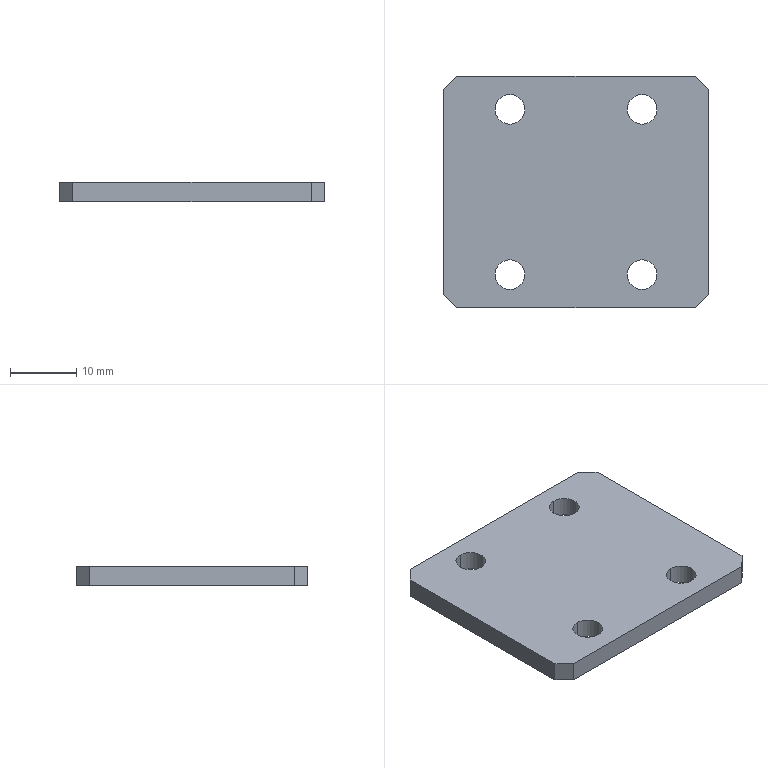Component | SolidWorks | 170423A4-RetainingPlate1-1 | 1 solid | 18 faces | box 40 x 35 x 3 mm | volume 3985 mm3 | plane 10 | cylinder 8 | commonest cylinder face diameters 4.5 x8
build123d program:
from build123d import *

# Parameters (mm, degrees)
SKETCH1_W                  = 35
SKETCH1_H                  = 40
BOSS_EXTRUDE1_DEPTH        = 3
F_4_5_4_5_DIAMETER_HOLE1_D = 4.5
CHAMFER1_SIZE              = 2


with BuildPart() as part:
    # Sketch1 → Boss-Extrude1 (new body)
    with BuildSketch(Plane.XY):
        Rectangle(SKETCH1_W, SKETCH1_H)
    extrude(amount=BOSS_EXTRUDE1_DEPTH)

    # 4.5 _4.5_ Diameter Hole1 (through all)
    with Locations(Plane.XY.offset(3)):
        with Locations((12.5, -10), (-12.5, 10), (-12.5, -10), (12.5, 10)):
            Hole(F_4_5_4_5_DIAMETER_HOLE1_D / 2)

    # Chamfer1
    chamfer1_edges = [part.edges().sort_by_distance(p)[0] for p in [
        (17.5, -20, 1.5),
        (-17.5, -20, 1.5),
        (-17.5, 20, 1.5),
        (17.5, 20, 1.5),
    ]]
    chamfer(chamfer1_edges, length=CHAMFER1_SIZE)


solid = part.part

# Placed as in the assembly
solid = solid.moved(Location((-1.246, -95.788, 406), (0, 0, 90)))
STEP:
#1=CARTESIAN_POINT('',(0.3446,-3.19,15.984));
#2=VERTEX_POINT('',#1);
#3=CARTESIAN_POINT('',(0.3446,-3.368,15.984));
#4=VERTEX_POINT('',#3);
#5=CARTESIAN_POINT('',(0.3446,-3.279,15.984));
#6=DIRECTION('',(0.,0.,1.));
#7=DIRECTION('',(0.,-1.,0.));
#8=AXIS2_PLACEMENT_3D('',#5,#6,#7);
#9=CIRCLE('',#8,0.08858);
#10=EDGE_CURVE('',#2,#4,#9,.T.);
#11=ORIENTED_EDGE('',*,*,#10,.F.);
#12=CARTESIAN_POINT('',(0.3446,-3.19,16.102));
#13=VERTEX_POINT('',#12);
#14=CARTESIAN_POINT('',(0.3446,-3.19,16.102));
#15=DIRECTION('',(0.,0.,1.));
#16=VECTOR('',#15,39.37);
#17=LINE('',#14,#16);
#18=EDGE_CURVE('',#2,#13,#17,.T.);
#19=ORIENTED_EDGE('',*,*,#18,.T.);
#20=CARTESIAN_POINT('',(0.3446,-3.368,16.102));
#21=VERTEX_POINT('',#20);
#22=CARTESIAN_POINT('',(0.3446,-3.279,16.102));
#23=DIRECTION('',(0.,0.,1.));
#24=DIRECTION('',(0.,-1.,0.));
#25=AXIS2_PLACEMENT_3D('',#22,#23,#24);
#26=CIRCLE('',#25,0.08858);
#27=EDGE_CURVE('',#13,#21,#26,.T.);
#28=ORIENTED_EDGE('',*,*,#27,.T.);
#29=CARTESIAN_POINT('',(0.3446,-3.368,16.102));
#30=DIRECTION('',(0.,0.,1.));
#31=VECTOR('',#30,39.37);
#32=LINE('',#29,#31);
#33=EDGE_CURVE('',#4,#21,#32,.T.);
#34=ORIENTED_EDGE('',*,*,#33,.F.);
#35=EDGE_LOOP('',(#11,#19,#28,#34));
#36=FACE_OUTER_BOUND('',#35,.T.);
#37=CARTESIAN_POINT('',(0.3446,-3.279,16.102));
#38=DIRECTION('',(0.,0.,1.));
#39=DIRECTION('',(0.,-1.,0.));
#40=AXIS2_PLACEMENT_3D('',#37,#38,#39);
#41=CYLINDRICAL_SURFACE('',#40,0.08858);
#42=ADVANCED_FACE('',(#36),#41,.F.);
#43=CARTESIAN_POINT('',(-0.4428,-3.19,15.984));
#44=VERTEX_POINT('',#43);
#45=CARTESIAN_POINT('',(-0.4428,-3.368,15.984));
#46=VERTEX_POINT('',#45);
#47=CARTESIAN_POINT('',(-0.4428,-3.279,15.984));
#48=DIRECTION('',(0.,0.,1.));
#49=DIRECTION('',(0.,-1.,0.));
#50=AXIS2_PLACEMENT_3D('',#47,#48,#49);
#51=CIRCLE('',#50,0.08858);
#52=EDGE_CURVE('',#44,#46,#51,.T.);
#53=ORIENTED_EDGE('',*,*,#52,.F.);
#54=CARTESIAN_POINT('',(-0.4428,-3.19,16.102));
#55=VERTEX_POINT('',#54);
#56=CARTESIAN_POINT('',(-0.4428,-3.19,16.102));
#57=DIRECTION('',(0.,0.,1.));
#58=VECTOR('',#57,39.37);
#59=LINE('',#56,#58);
#60=EDGE_CURVE('',#44,#55,#59,.T.);
#61=ORIENTED_EDGE('',*,*,#60,.T.);
#62=CARTESIAN_POINT('',(-0.4428,-3.368,16.102));
#63=VERTEX_POINT('',#62);
#64=CARTESIAN_POINT('',(-0.4428,-3.279,16.102));
#65=DIRECTION('',(0.,0.,1.));
#66=DIRECTION('',(0.,-1.,0.));
#67=AXIS2_PLACEMENT_3D('',#64,#65,#66);
#68=CIRCLE('',#67,0.08858);
#69=EDGE_CURVE('',#55,#63,#68,.T.);
#70=ORIENTED_EDGE('',*,*,#69,.T.);
#71=CARTESIAN_POINT('',(-0.4428,-3.368,16.102));
#72=DIRECTION('',(0.,0.,1.));
#73=VECTOR('',#72,39.37);
#74=LINE('',#71,#73);
#75=EDGE_CURVE('',#46,#63,#74,.T.);
#76=ORIENTED_EDGE('',*,*,#75,.F.);
#77=EDGE_LOOP('',(#53,#61,#70,#76));
#78=FACE_OUTER_BOUND('',#77,.T.);
#79=CARTESIAN_POINT('',(-0.4428,-3.279,16.102));
#80=DIRECTION('',(0.,0.,1.));
#81=DIRECTION('',(0.,-1.,0.));
#82=AXIS2_PLACEMENT_3D('',#79,#80,#81);
#83=CYLINDRICAL_SURFACE('',#82,0.08858);
#84=ADVANCED_FACE('',(#78),#83,.F.);
#85=CARTESIAN_POINT('',(0.3446,-4.175,15.984));
#86=VERTEX_POINT('',#85);
#87=CARTESIAN_POINT('',(0.3446,-4.352,15.984));
#88=VERTEX_POINT('',#87);
#89=CARTESIAN_POINT('',(0.3446,-4.263,15.984));
#90=DIRECTION('',(0.,0.,1.));
#91=DIRECTION('',(0.,-1.,0.));
#92=AXIS2_PLACEMENT_3D('',#89,#90,#91);
#93=CIRCLE('',#92,0.08858);
#94=EDGE_CURVE('',#86,#88,#93,.T.);
#95=ORIENTED_EDGE('',*,*,#94,.F.);
#96=CARTESIAN_POINT('',(0.3446,-4.175,16.102));
#97=VERTEX_POINT('',#96);
#98=CARTESIAN_POINT('',(0.3446,-4.175,16.102));
#99=DIRECTION('',(0.,0.,1.));
#100=VECTOR('',#99,39.37);
#101=LINE('',#98,#100);
#102=EDGE_CURVE('',#86,#97,#101,.T.);
#103=ORIENTED_EDGE('',*,*,#102,.T.);
#104=CARTESIAN_POINT('',(0.3446,-4.352,16.102));
#105=VERTEX_POINT('',#104);
#106=CARTESIAN_POINT('',(0.3446,-4.263,16.102));
#107=DIRECTION('',(0.,0.,1.));
#108=DIRECTION('',(0.,-1.,0.));
#109=AXIS2_PLACEMENT_3D('',#106,#107,#108);
#110=CIRCLE('',#109,0.08858);
#111=EDGE_CURVE('',#97,#105,#110,.T.);
#112=ORIENTED_EDGE('',*,*,#111,.T.);
#113=CARTESIAN_POINT('',(0.3446,-4.352,16.102));
#114=DIRECTION('',(0.,0.,1.));
#115=VECTOR('',#114,39.37);
#116=LINE('',#113,#115);
#117=EDGE_CURVE('',#88,#105,#116,.T.);
#118=ORIENTED_EDGE('',*,*,#117,.F.);
#119=EDGE_LOOP('',(#95,#103,#112,#118));
#120=FACE_OUTER_BOUND('',#119,.T.);
#121=CARTESIAN_POINT('',(0.3446,-4.263,16.102));
#122=DIRECTION('',(0.,0.,1.));
#123=DIRECTION('',(0.,-1.,0.));
#124=AXIS2_PLACEMENT_3D('',#121,#122,#123);
#125=CYLINDRICAL_SURFACE('',#124,0.08858);
#126=ADVANCED_FACE('',(#120),#125,.F.);
#127=CARTESIAN_POINT('',(-0.4428,-4.175,15.984));
#128=VERTEX_POINT('',#127);
#129=CARTESIAN_POINT('',(-0.4428,-4.352,15.984));
#130=VERTEX_POINT('',#129);
#131=CARTESIAN_POINT('',(-0.4428,-4.263,15.984));
#132=DIRECTION('',(0.,0.,1.));
#133=DIRECTION('',(0.,-1.,0.));
#134=AXIS2_PLACEMENT_3D('',#131,#132,#133);
#135=CIRCLE('',#134,0.08858);
#136=EDGE_CURVE('',#128,#130,#135,.T.);
#137=ORIENTED_EDGE('',*,*,#136,.F.);
#138=CARTESIAN_POINT('',(-0.4428,-4.175,16.102));
#139=VERTEX_POINT('',#138);
#140=CARTESIAN_POINT('',(-0.4428,-4.175,16.102));
#141=DIRECTION('',(0.,0.,1.));
#142=VECTOR('',#141,39.37);
#143=LINE('',#140,#142);
#144=EDGE_CURVE('',#128,#139,#143,.T.);
#145=ORIENTED_EDGE('',*,*,#144,.T.);
#146=CARTESIAN_POINT('',(-0.4428,-4.352,16.102));
#147=VERTEX_POINT('',#146);
#148=CARTESIAN_POINT('',(-0.4428,-4.263,16.102));
#149=DIRECTION('',(0.,0.,1.));
#150=DIRECTION('',(0.,-1.,0.));
#151=AXIS2_PLACEMENT_3D('',#148,#149,#150);
#152=CIRCLE('',#151,0.08858);
#153=EDGE_CURVE('',#139,#147,#152,.T.);
#154=ORIENTED_EDGE('',*,*,#153,.T.);
#155=CARTESIAN_POINT('',(-0.4428,-4.352,16.102));
#156=DIRECTION('',(0.,0.,1.));
#157=VECTOR('',#156,39.37);
#158=LINE('',#155,#157);
#159=EDGE_CURVE('',#130,#147,#158,.T.);
#160=ORIENTED_EDGE('',*,*,#159,.F.);
#161=EDGE_LOOP('',(#137,#145,#154,#160));
#162=FACE_OUTER_BOUND('',#161,.T.);
#163=CARTESIAN_POINT('',(-0.4428,-4.263,16.102));
#164=DIRECTION('',(0.,0.,1.));
#165=DIRECTION('',(0.,-1.,0.));
#166=AXIS2_PLACEMENT_3D('',#163,#164,#165);
#167=CYLINDRICAL_SURFACE('',#166,0.08858);
#168=ADVANCED_FACE('',(#162),#167,.F.);
#169=CARTESIAN_POINT('',(-0.7577,-4.46,16.102));
#170=VERTEX_POINT('',#169);
#171=CARTESIAN_POINT('',(0.6596,-4.46,16.102));
#172=VERTEX_POINT('',#171);
#173=CARTESIAN_POINT('',(0.7383,-4.46,16.102));
#174=DIRECTION('',(1.,0.,0.));
#175=VECTOR('',#174,39.37);
#176=LINE('',#173,#175);
#177=EDGE_CURVE('',#170,#172,#176,.T.);
#178=ORIENTED_EDGE('',*,*,#177,.F.);
#179=CARTESIAN_POINT('',(-0.7577,-4.46,15.984));
#180=VERTEX_POINT('',#179);
#181=CARTESIAN_POINT('',(-0.7577,-4.46,16.102));
#182=DIRECTION('',(0.,0.,-1.));
#183=VECTOR('',#182,39.37);
#184=LINE('',#181,#183);
#185=EDGE_CURVE('',#170,#180,#184,.T.);
#186=ORIENTED_EDGE('',*,*,#185,.T.);
#187=CARTESIAN_POINT('',(0.6596,-4.46,15.984));
#188=VERTEX_POINT('',#187);
#189=CARTESIAN_POINT('',(0.7383,-4.46,15.984));
#190=DIRECTION('',(1.,0.,0.));
#191=VECTOR('',#190,39.37);
#192=LINE('',#189,#191);
#193=EDGE_CURVE('',#180,#188,#192,.T.);
#194=ORIENTED_EDGE('',*,*,#193,.T.);
#195=CARTESIAN_POINT('',(0.6596,-4.46,16.102));
#196=DIRECTION('',(0.,0.,1.));
#197=VECTOR('',#196,39.37);
#198=LINE('',#195,#197);
#199=EDGE_CURVE('',#188,#172,#198,.T.);
#200=ORIENTED_EDGE('',*,*,#199,.T.);
#201=EDGE_LOOP('',(#178,#186,#194,#200));
#202=FACE_OUTER_BOUND('',#201,.T.);
#203=CARTESIAN_POINT('',(0.7383,-4.46,16.102));
#204=DIRECTION('',(-0.,1.,0.));
#205=DIRECTION('',(-1.,-0.,0.));
#206=AXIS2_PLACEMENT_3D('',#203,#204,#205);
#207=PLANE('',#206);
#208=ADVANCED_FACE('',(#202),#207,.F.);
#209=CARTESIAN_POINT('',(0.7383,-4.381,15.984));
#210=VERTEX_POINT('',#209);
#211=CARTESIAN_POINT('',(0.7383,-3.161,15.984));
#212=VERTEX_POINT('',#211);
#213=CARTESIAN_POINT('',(0.7383,-3.082,15.984));
#214=DIRECTION('',(0.,1.,0.));
#215=VECTOR('',#214,39.37);
#216=LINE('',#213,#215);
#217=EDGE_CURVE('',#210,#212,#216,.T.);
#218=ORIENTED_EDGE('',*,*,#217,.T.);
#219=CARTESIAN_POINT('',(0.7383,-3.161,16.102));
#220=VERTEX_POINT('',#219);
#221=CARTESIAN_POINT('',(0.7383,-3.161,16.102));
#222=DIRECTION('',(0.,0.,1.));
#223=VECTOR('',#222,39.37);
#224=LINE('',#221,#223);
#225=EDGE_CURVE('',#212,#220,#224,.T.);
#226=ORIENTED_EDGE('',*,*,#225,.T.);
#227=CARTESIAN_POINT('',(0.7383,-4.381,16.102));
#228=VERTEX_POINT('',#227);
#229=CARTESIAN_POINT('',(0.7383,-3.082,16.102));
#230=DIRECTION('',(0.,1.,0.));
#231=VECTOR('',#230,39.37);
#232=LINE('',#229,#231);
#233=EDGE_CURVE('',#228,#220,#232,.T.);
#234=ORIENTED_EDGE('',*,*,#233,.F.);
#235=CARTESIAN_POINT('',(0.7383,-4.381,16.102));
#236=DIRECTION('',(0.,0.,-1.));
#237=VECTOR('',#236,39.37);
#238=LINE('',#235,#237);
#239=EDGE_CURVE('',#228,#210,#238,.T.);
#240=ORIENTED_EDGE('',*,*,#239,.T.);
#241=EDGE_LOOP('',(#218,#226,#234,#240));
#242=FACE_OUTER_BOUND('',#241,.T.);
#243=CARTESIAN_POINT('',(0.7383,-3.082,16.102));
#244=DIRECTION('',(-1.,0.,0.));
#245=DIRECTION('',(0.,0.,-1.));
#246=AXIS2_PLACEMENT_3D('',#243,#244,#245);
#247=PLANE('',#246);
#248=ADVANCED_FACE('',(#242),#247,.F.);
#249=CARTESIAN_POINT('',(0.6596,-3.082,15.984));
#250=VERTEX_POINT('',#249);
#251=CARTESIAN_POINT('',(-0.7577,-3.082,15.984));
#252=VERTEX_POINT('',#251);
#253=CARTESIAN_POINT('',(0.7383,-3.082,15.984));
#254=DIRECTION('',(-1.,-0.,0.));
#255=VECTOR('',#254,39.37);
#256=LINE('',#253,#255);
#257=EDGE_CURVE('',#250,#252,#256,.T.);
#258=ORIENTED_EDGE('',*,*,#257,.T.);
#259=CARTESIAN_POINT('',(-0.7577,-3.082,16.102));
#260=VERTEX_POINT('',#259);
#261=CARTESIAN_POINT('',(-0.7577,-3.082,16.102));
#262=DIRECTION('',(0.,0.,1.));
#263=VECTOR('',#262,39.37);
#264=LINE('',#261,#263);
#265=EDGE_CURVE('',#252,#260,#264,.T.);
#266=ORIENTED_EDGE('',*,*,#265,.T.);
#267=CARTESIAN_POINT('',(0.6596,-3.082,16.102));
#268=VERTEX_POINT('',#267);
#269=CARTESIAN_POINT('',(0.7383,-3.082,16.102));
#270=DIRECTION('',(-1.,-0.,0.));
#271=VECTOR('',#270,39.37);
#272=LINE('',#269,#271);
#273=EDGE_CURVE('',#268,#260,#272,.T.);
#274=ORIENTED_EDGE('',*,*,#273,.F.);
#275=CARTESIAN_POINT('',(0.6596,-3.082,16.102));
#276=DIRECTION('',(0.,0.,-1.));
#277=VECTOR('',#276,39.37);
#278=LINE('',#275,#277);
#279=EDGE_CURVE('',#268,#250,#278,.T.);
#280=ORIENTED_EDGE('',*,*,#279,.T.);
#281=EDGE_LOOP('',(#258,#266,#274,#280));
#282=FACE_OUTER_BOUND('',#281,.T.);
#283=CARTESIAN_POINT('',(0.7383,-3.082,16.102));
#284=DIRECTION('',(0.,-1.,0.));
#285=DIRECTION('',(1.,0.,0.));
#286=AXIS2_PLACEMENT_3D('',#283,#284,#285);
#287=PLANE('',#286);
#288=ADVANCED_FACE('',(#282),#287,.F.);
#289=CARTESIAN_POINT('',(-0.8365,-3.161,16.102));
#290=VERTEX_POINT('',#289);
#291=CARTESIAN_POINT('',(-0.8365,-4.381,16.102));
#292=VERTEX_POINT('',#291);
#293=CARTESIAN_POINT('',(-0.8365,-3.082,16.102));
#294=DIRECTION('',(0.,-1.,0.));
#295=VECTOR('',#294,39.37);
#296=LINE('',#293,#295);
#297=EDGE_CURVE('',#290,#292,#296,.T.);
#298=ORIENTED_EDGE('',*,*,#297,.F.);
#299=CARTESIAN_POINT('',(-0.8365,-3.161,15.984));
#300=VERTEX_POINT('',#299);
#301=CARTESIAN_POINT('',(-0.8365,-3.161,16.102));
#302=DIRECTION('',(0.,0.,-1.));
#303=VECTOR('',#302,39.37);
#304=LINE('',#301,#303);
#305=EDGE_CURVE('',#290,#300,#304,.T.);
#306=ORIENTED_EDGE('',*,*,#305,.T.);
#307=CARTESIAN_POINT('',(-0.8365,-4.381,15.984));
#308=VERTEX_POINT('',#307);
#309=CARTESIAN_POINT('',(-0.8365,-3.082,15.984));
#310=DIRECTION('',(0.,-1.,0.));
#311=VECTOR('',#310,39.37);
#312=LINE('',#309,#311);
#313=EDGE_CURVE('',#300,#308,#312,.T.);
#314=ORIENTED_EDGE('',*,*,#313,.T.);
#315=CARTESIAN_POINT('',(-0.8365,-4.381,16.102));
#316=DIRECTION('',(0.,0.,1.));
#317=VECTOR('',#316,39.37);
#318=LINE('',#315,#317);
#319=EDGE_CURVE('',#308,#292,#318,.T.);
#320=ORIENTED_EDGE('',*,*,#319,.T.);
#321=EDGE_LOOP('',(#298,#306,#314,#320));
#322=FACE_OUTER_BOUND('',#321,.T.);
#323=CARTESIAN_POINT('',(-0.8365,-3.082,16.102));
#324=DIRECTION('',(1.,0.,0.));
#325=DIRECTION('',(0.,0.,1.));
#326=AXIS2_PLACEMENT_3D('',#323,#324,#325);
#327=PLANE('',#326);
#328=ADVANCED_FACE('',(#322),#327,.F.);
#329=CARTESIAN_POINT('',(0.3446,-3.279,16.102));
#330=DIRECTION('',(0.,0.,1.));
#331=DIRECTION('',(0.,-1.,0.));
#332=AXIS2_PLACEMENT_3D('',#329,#330,#331);
#333=CIRCLE('',#332,0.08858);
#334=EDGE_CURVE('',#21,#13,#333,.T.);
#335=ORIENTED_EDGE('',*,*,#334,.F.);
#336=ORIENTED_EDGE('',*,*,#27,.F.);
#337=EDGE_LOOP('',(#335,#336));
#338=FACE_BOUND('',#337,.T.);
#339=CARTESIAN_POINT('',(-0.4428,-3.279,16.102));
#340=DIRECTION('',(0.,0.,1.));
#341=DIRECTION('',(0.,-1.,0.));
#342=AXIS2_PLACEMENT_3D('',#339,#340,#341);
#343=CIRCLE('',#342,0.08858);
#344=EDGE_CURVE('',#63,#55,#343,.T.);
#345=ORIENTED_EDGE('',*,*,#344,.F.);
#346=ORIENTED_EDGE('',*,*,#69,.F.);
#347=EDGE_LOOP('',(#345,#346));
#348=FACE_BOUND('',#347,.T.);
#349=CARTESIAN_POINT('',(0.3446,-4.263,16.102));
#350=DIRECTION('',(0.,0.,1.));
#351=DIRECTION('',(0.,-1.,0.));
#352=AXIS2_PLACEMENT_3D('',#349,#350,#351);
#353=CIRCLE('',#352,0.08858);
#354=EDGE_CURVE('',#105,#97,#353,.T.);
#355=ORIENTED_EDGE('',*,*,#354,.F.);
#356=ORIENTED_EDGE('',*,*,#111,.F.);
#357=EDGE_LOOP('',(#355,#356));
#358=FACE_BOUND('',#357,.T.);
#359=CARTESIAN_POINT('',(-0.4428,-4.263,16.102));
#360=DIRECTION('',(0.,0.,1.));
#361=DIRECTION('',(0.,-1.,0.));
#362=AXIS2_PLACEMENT_3D('',#359,#360,#361);
#363=CIRCLE('',#362,0.08858);
#364=EDGE_CURVE('',#147,#139,#363,.T.);
#365=ORIENTED_EDGE('',*,*,#364,.F.);
#366=ORIENTED_EDGE('',*,*,#153,.F.);
#367=EDGE_LOOP('',(#365,#366));
#368=FACE_BOUND('',#367,.T.);
#369=ORIENTED_EDGE('',*,*,#273,.T.);
#370=CARTESIAN_POINT('',(-0.7479,-3.072,16.102));
#371=DIRECTION('',(-0.7071,-0.7071,0.));
#372=VECTOR('',#371,39.37);
#373=LINE('',#370,#372);
#374=EDGE_CURVE('',#260,#290,#373,.T.);
#375=ORIENTED_EDGE('',*,*,#374,.T.);
#376=ORIENTED_EDGE('',*,*,#297,.T.);
#377=CARTESIAN_POINT('',(-0.7479,-4.47,16.102));
#378=DIRECTION('',(0.7071,-0.7071,0.));
#379=VECTOR('',#378,39.37);
#380=LINE('',#377,#379);
#381=EDGE_CURVE('',#292,#170,#380,.T.);
#382=ORIENTED_EDGE('',*,*,#381,.T.);
#383=ORIENTED_EDGE('',*,*,#177,.T.);
#384=CARTESIAN_POINT('',(0.6497,-4.47,16.102));
#385=DIRECTION('',(0.7071,0.7071,0.));
#386=VECTOR('',#385,39.37);
#387=LINE('',#384,#386);
#388=EDGE_CURVE('',#172,#228,#387,.T.);
#389=ORIENTED_EDGE('',*,*,#388,.T.);
#390=ORIENTED_EDGE('',*,*,#233,.T.);
#391=CARTESIAN_POINT('',(0.6497,-3.072,16.102));
#392=DIRECTION('',(-0.7071,0.7071,0.));
#393=VECTOR('',#392,39.37);
#394=LINE('',#391,#393);
#395=EDGE_CURVE('',#220,#268,#394,.T.);
#396=ORIENTED_EDGE('',*,*,#395,.T.);
#397=EDGE_LOOP('',(#369,#375,#376,#382,#383,#389,#390,#396));
#398=FACE_OUTER_BOUND('',#397,.T.);
#399=CARTESIAN_POINT('',(-0.04907,-3.771,16.102));
#400=DIRECTION('',(0.,0.,1.));
#401=DIRECTION('',(0.,-1.,0.));
#402=AXIS2_PLACEMENT_3D('',#399,#400,#401);
#403=PLANE('',#402);
#404=ADVANCED_FACE('',(#338,#348,#358,#368,#398),#403,.T.);
#405=CARTESIAN_POINT('',(0.3446,-3.279,15.984));
#406=DIRECTION('',(0.,0.,1.));
#407=DIRECTION('',(0.,-1.,0.));
#408=AXIS2_PLACEMENT_3D('',#405,#406,#407);
#409=CIRCLE('',#408,0.08858);
#410=EDGE_CURVE('',#4,#2,#409,.T.);
#411=ORIENTED_EDGE('',*,*,#410,.T.);
#412=ORIENTED_EDGE('',*,*,#10,.T.);
#413=EDGE_LOOP('',(#411,#412));
#414=FACE_BOUND('',#413,.T.);
#415=CARTESIAN_POINT('',(-0.4428,-3.279,15.984));
#416=DIRECTION('',(0.,0.,1.));
#417=DIRECTION('',(0.,-1.,0.));
#418=AXIS2_PLACEMENT_3D('',#415,#416,#417);
#419=CIRCLE('',#418,0.08858);
#420=EDGE_CURVE('',#46,#44,#419,.T.);
#421=ORIENTED_EDGE('',*,*,#420,.T.);
#422=ORIENTED_EDGE('',*,*,#52,.T.);
#423=EDGE_LOOP('',(#421,#422));
#424=FACE_BOUND('',#423,.T.);
#425=CARTESIAN_POINT('',(0.3446,-4.263,15.984));
#426=DIRECTION('',(0.,0.,1.));
#427=DIRECTION('',(0.,-1.,0.));
#428=AXIS2_PLACEMENT_3D('',#425,#426,#427);
#429=CIRCLE('',#428,0.08858);
#430=EDGE_CURVE('',#88,#86,#429,.T.);
#431=ORIENTED_EDGE('',*,*,#430,.T.);
#432=ORIENTED_EDGE('',*,*,#94,.T.);
#433=EDGE_LOOP('',(#431,#432));
#434=FACE_BOUND('',#433,.T.);
#435=CARTESIAN_POINT('',(-0.4428,-4.263,15.984));
#436=DIRECTION('',(0.,0.,1.));
#437=DIRECTION('',(0.,-1.,0.));
#438=AXIS2_PLACEMENT_3D('',#435,#436,#437);
#439=CIRCLE('',#438,0.08858);
#440=EDGE_CURVE('',#130,#128,#439,.T.);
#441=ORIENTED_EDGE('',*,*,#440,.T.);
#442=ORIENTED_EDGE('',*,*,#136,.T.);
#443=EDGE_LOOP('',(#441,#442));
#444=FACE_BOUND('',#443,.T.);
#445=ORIENTED_EDGE('',*,*,#313,.F.);
#446=CARTESIAN_POINT('',(-0.8365,-3.161,15.984));
#447=DIRECTION('',(0.7071,0.7071,0.));
#448=VECTOR('',#447,39.37);
#449=LINE('',#446,#448);
#450=EDGE_CURVE('',#300,#252,#449,.T.);
#451=ORIENTED_EDGE('',*,*,#450,.T.);
#452=ORIENTED_EDGE('',*,*,#257,.F.);
#453=CARTESIAN_POINT('',(0.6596,-3.082,15.984));
#454=DIRECTION('',(0.7071,-0.7071,0.));
#455=VECTOR('',#454,39.37);
#456=LINE('',#453,#455);
#457=EDGE_CURVE('',#250,#212,#456,.T.);
#458=ORIENTED_EDGE('',*,*,#457,.T.);
#459=ORIENTED_EDGE('',*,*,#217,.F.);
#460=CARTESIAN_POINT('',(0.7383,-4.381,15.984));
#461=DIRECTION('',(-0.7071,-0.7071,0.));
#462=VECTOR('',#461,39.37);
#463=LINE('',#460,#462);
#464=EDGE_CURVE('',#210,#188,#463,.T.);
#465=ORIENTED_EDGE('',*,*,#464,.T.);
#466=ORIENTED_EDGE('',*,*,#193,.F.);
#467=CARTESIAN_POINT('',(-0.7577,-4.46,15.984));
#468=DIRECTION('',(-0.7071,0.7071,0.));
#469=VECTOR('',#468,39.37);
#470=LINE('',#467,#469);
#471=EDGE_CURVE('',#180,#308,#470,.T.);
#472=ORIENTED_EDGE('',*,*,#471,.T.);
#473=EDGE_LOOP('',(#445,#451,#452,#458,#459,#465,#466,#472));
#474=FACE_OUTER_BOUND('',#473,.T.);
#475=CARTESIAN_POINT('',(-0.04907,-3.771,15.984));
#476=DIRECTION('',(0.,0.,1.));
#477=DIRECTION('',(0.,-1.,0.));
#478=AXIS2_PLACEMENT_3D('',#475,#476,#477);
#479=PLANE('',#478);
#480=ADVANCED_FACE('',(#414,#424,#434,#444,#474),#479,.F.);
#481=ORIENTED_EDGE('',*,*,#144,.F.);
#482=ORIENTED_EDGE('',*,*,#440,.F.);
#483=ORIENTED_EDGE('',*,*,#159,.T.);
#484=ORIENTED_EDGE('',*,*,#364,.T.);
#485=EDGE_LOOP('',(#481,#482,#483,#484));
#486=FACE_OUTER_BOUND('',#485,.T.);
#487=CARTESIAN_POINT('',(-0.4428,-4.263,16.102));
#488=DIRECTION('',(0.,0.,1.));
#489=DIRECTION('',(0.,-1.,0.));
#490=AXIS2_PLACEMENT_3D('',#487,#488,#489);
#491=CYLINDRICAL_SURFACE('',#490,0.08858);
#492=ADVANCED_FACE('',(#486),#491,.F.);
#493=ORIENTED_EDGE('',*,*,#102,.F.);
#494=ORIENTED_EDGE('',*,*,#430,.F.);
#495=ORIENTED_EDGE('',*,*,#117,.T.);
#496=ORIENTED_EDGE('',*,*,#354,.T.);
#497=EDGE_LOOP('',(#493,#494,#495,#496));
#498=FACE_OUTER_BOUND('',#497,.T.);
#499=CARTESIAN_POINT('',(0.3446,-4.263,16.102));
#500=DIRECTION('',(0.,0.,1.));
#501=DIRECTION('',(0.,-1.,0.));
#502=AXIS2_PLACEMENT_3D('',#499,#500,#501);
#503=CYLINDRICAL_SURFACE('',#502,0.08858);
#504=ADVANCED_FACE('',(#498),#503,.F.);
#505=ORIENTED_EDGE('',*,*,#60,.F.);
#506=ORIENTED_EDGE('',*,*,#420,.F.);
#507=ORIENTED_EDGE('',*,*,#75,.T.);
#508=ORIENTED_EDGE('',*,*,#344,.T.);
#509=EDGE_LOOP('',(#505,#506,#507,#508));
#510=FACE_OUTER_BOUND('',#509,.T.);
#511=CARTESIAN_POINT('',(-0.4428,-3.279,16.102));
#512=DIRECTION('',(0.,0.,1.));
#513=DIRECTION('',(0.,-1.,0.));
#514=AXIS2_PLACEMENT_3D('',#511,#512,#513);
#515=CYLINDRICAL_SURFACE('',#514,0.08858);
#516=ADVANCED_FACE('',(#510),#515,.F.);
#517=ORIENTED_EDGE('',*,*,#18,.F.);
#518=ORIENTED_EDGE('',*,*,#410,.F.);
#519=ORIENTED_EDGE('',*,*,#33,.T.);
#520=ORIENTED_EDGE('',*,*,#334,.T.);
#521=EDGE_LOOP('',(#517,#518,#519,#520));
#522=FACE_OUTER_BOUND('',#521,.T.);
#523=CARTESIAN_POINT('',(0.3446,-3.279,16.102));
#524=DIRECTION('',(0.,0.,1.));
#525=DIRECTION('',(0.,-1.,0.));
#526=AXIS2_PLACEMENT_3D('',#523,#524,#525);
#527=CYLINDRICAL_SURFACE('',#526,0.08858);
#528=ADVANCED_FACE('',(#522),#527,.F.);
#529=ORIENTED_EDGE('',*,*,#374,.F.);
#530=ORIENTED_EDGE('',*,*,#265,.F.);
#531=ORIENTED_EDGE('',*,*,#450,.F.);
#532=ORIENTED_EDGE('',*,*,#305,.F.);
#533=EDGE_LOOP('',(#529,#530,#531,#532));
#534=FACE_OUTER_BOUND('',#533,.T.);
#535=CARTESIAN_POINT('',(-0.8365,-3.161,16.102));
#536=DIRECTION('',(0.7071,-0.7071,0.));
#537=DIRECTION('',(0.,0.,-1.));
#538=AXIS2_PLACEMENT_3D('',#535,#536,#537);
#539=PLANE('',#538);
#540=ADVANCED_FACE('',(#534),#539,.F.);
#541=ORIENTED_EDGE('',*,*,#395,.F.);
#542=ORIENTED_EDGE('',*,*,#225,.F.);
#543=ORIENTED_EDGE('',*,*,#457,.F.);
#544=ORIENTED_EDGE('',*,*,#279,.F.);
#545=EDGE_LOOP('',(#541,#542,#543,#544));
#546=FACE_OUTER_BOUND('',#545,.T.);
#547=CARTESIAN_POINT('',(0.6596,-3.082,16.102));
#548=DIRECTION('',(-0.7071,-0.7071,0.));
#549=DIRECTION('',(0.,0.,-1.));
#550=AXIS2_PLACEMENT_3D('',#547,#548,#549);
#551=PLANE('',#550);
#552=ADVANCED_FACE('',(#546),#551,.F.);
#553=ORIENTED_EDGE('',*,*,#381,.F.);
#554=ORIENTED_EDGE('',*,*,#319,.F.);
#555=ORIENTED_EDGE('',*,*,#471,.F.);
#556=ORIENTED_EDGE('',*,*,#185,.F.);
#557=EDGE_LOOP('',(#553,#554,#555,#556));
#558=FACE_OUTER_BOUND('',#557,.T.);
#559=CARTESIAN_POINT('',(-0.7577,-4.46,16.102));
#560=DIRECTION('',(0.7071,0.7071,0.));
#561=DIRECTION('',(0.,0.,-1.));
#562=AXIS2_PLACEMENT_3D('',#559,#560,#561);
#563=PLANE('',#562);
#564=ADVANCED_FACE('',(#558),#563,.F.);
#565=ORIENTED_EDGE('',*,*,#388,.F.);
#566=ORIENTED_EDGE('',*,*,#199,.F.);
#567=ORIENTED_EDGE('',*,*,#464,.F.);
#568=ORIENTED_EDGE('',*,*,#239,.F.);
#569=EDGE_LOOP('',(#565,#566,#567,#568));
#570=FACE_OUTER_BOUND('',#569,.T.);
#571=CARTESIAN_POINT('',(0.7383,-4.381,16.102));
#572=DIRECTION('',(-0.7071,0.7071,0.));
#573=DIRECTION('',(0.,0.,-1.));
#574=AXIS2_PLACEMENT_3D('',#571,#572,#573);
#575=PLANE('',#574);
#576=ADVANCED_FACE('',(#570),#575,.F.);
#577=CLOSED_SHELL('',(#42,#84,#126,#168,#208,#248,#288,#328,#404,#480,#492,#504,#516,#528,#540,#552,#564,#576));
#578=MANIFOLD_SOLID_BREP('',#577);
#579=CARTESIAN_POINT('',(0.,0.,0.));
#580=DIRECTION('',(0.,0.,1.));
#581=DIRECTION('',(1.,0.,0.));
#582=AXIS2_PLACEMENT_3D('',#579,#580,#581);
#583=(LENGTH_UNIT()NAMED_UNIT(*)SI_UNIT($,.METRE.));
#584=LENGTH_MEASURE_WITH_UNIT(LENGTH_MEASURE(0.0254),#583);
#585=DIMENSIONAL_EXPONENTS(1.,0.,0.,0.,0.,0.,0.);
#586=(CONVERSION_BASED_UNIT('',#584)LENGTH_UNIT()NAMED_UNIT(#585));
#587=UNCERTAINTY_MEASURE_WITH_UNIT(LENGTH_MEASURE(0.00001),#586,'','');
#588=(NAMED_UNIT(*)PLANE_ANGLE_UNIT()SI_UNIT($,.RADIAN.));
#589=(NAMED_UNIT(*)SI_UNIT($,.STERADIAN.)SOLID_ANGLE_UNIT());
#590=(GEOMETRIC_REPRESENTATION_CONTEXT(3)GLOBAL_UNCERTAINTY_ASSIGNED_CONTEXT((#587))GLOBAL_UNIT_ASSIGNED_CONTEXT((#586,#588,#589))REPRESENTATION_CONTEXT('',''));
#591=ADVANCED_BREP_SHAPE_REPRESENTATION('',(#578,#582),#590);
#592=COLOUR_RGB('',0.7922,0.8196,0.9333);
#593=FILL_AREA_STYLE_COLOUR('',#592);
#594=FILL_AREA_STYLE('',(#593));
#595=SURFACE_STYLE_FILL_AREA(#594);
#596=SURFACE_SIDE_STYLE('',(#595));
#597=SURFACE_STYLE_USAGE(.BOTH.,#596);
#598=PRESENTATION_STYLE_ASSIGNMENT((#597));
#599=STYLED_ITEM('',(#598),#578);
#600=PRESENTATION_LAYER_ASSIGNMENT('','',(#599));
#601=(LENGTH_UNIT()NAMED_UNIT(*)SI_UNIT($,.METRE.));
#602=LENGTH_MEASURE_WITH_UNIT(LENGTH_MEASURE(0.0254),#601);
#603=DIMENSIONAL_EXPONENTS(1.,0.,0.,0.,0.,0.,0.);
#604=(CONVERSION_BASED_UNIT('',#602)LENGTH_UNIT()NAMED_UNIT(#603));
#605=UNCERTAINTY_MEASURE_WITH_UNIT(LENGTH_MEASURE(0.00001),#604,'','');
#606=(NAMED_UNIT(*)PLANE_ANGLE_UNIT()SI_UNIT($,.RADIAN.));
#607=(NAMED_UNIT(*)SI_UNIT($,.STERADIAN.)SOLID_ANGLE_UNIT());
#608=(GEOMETRIC_REPRESENTATION_CONTEXT(3)GLOBAL_UNCERTAINTY_ASSIGNED_CONTEXT((#605))GLOBAL_UNIT_ASSIGNED_CONTEXT((#604,#606,#607))REPRESENTATION_CONTEXT('',''));
#609=MECHANICAL_DESIGN_GEOMETRIC_PRESENTATION_REPRESENTATION('',(#599),#608);